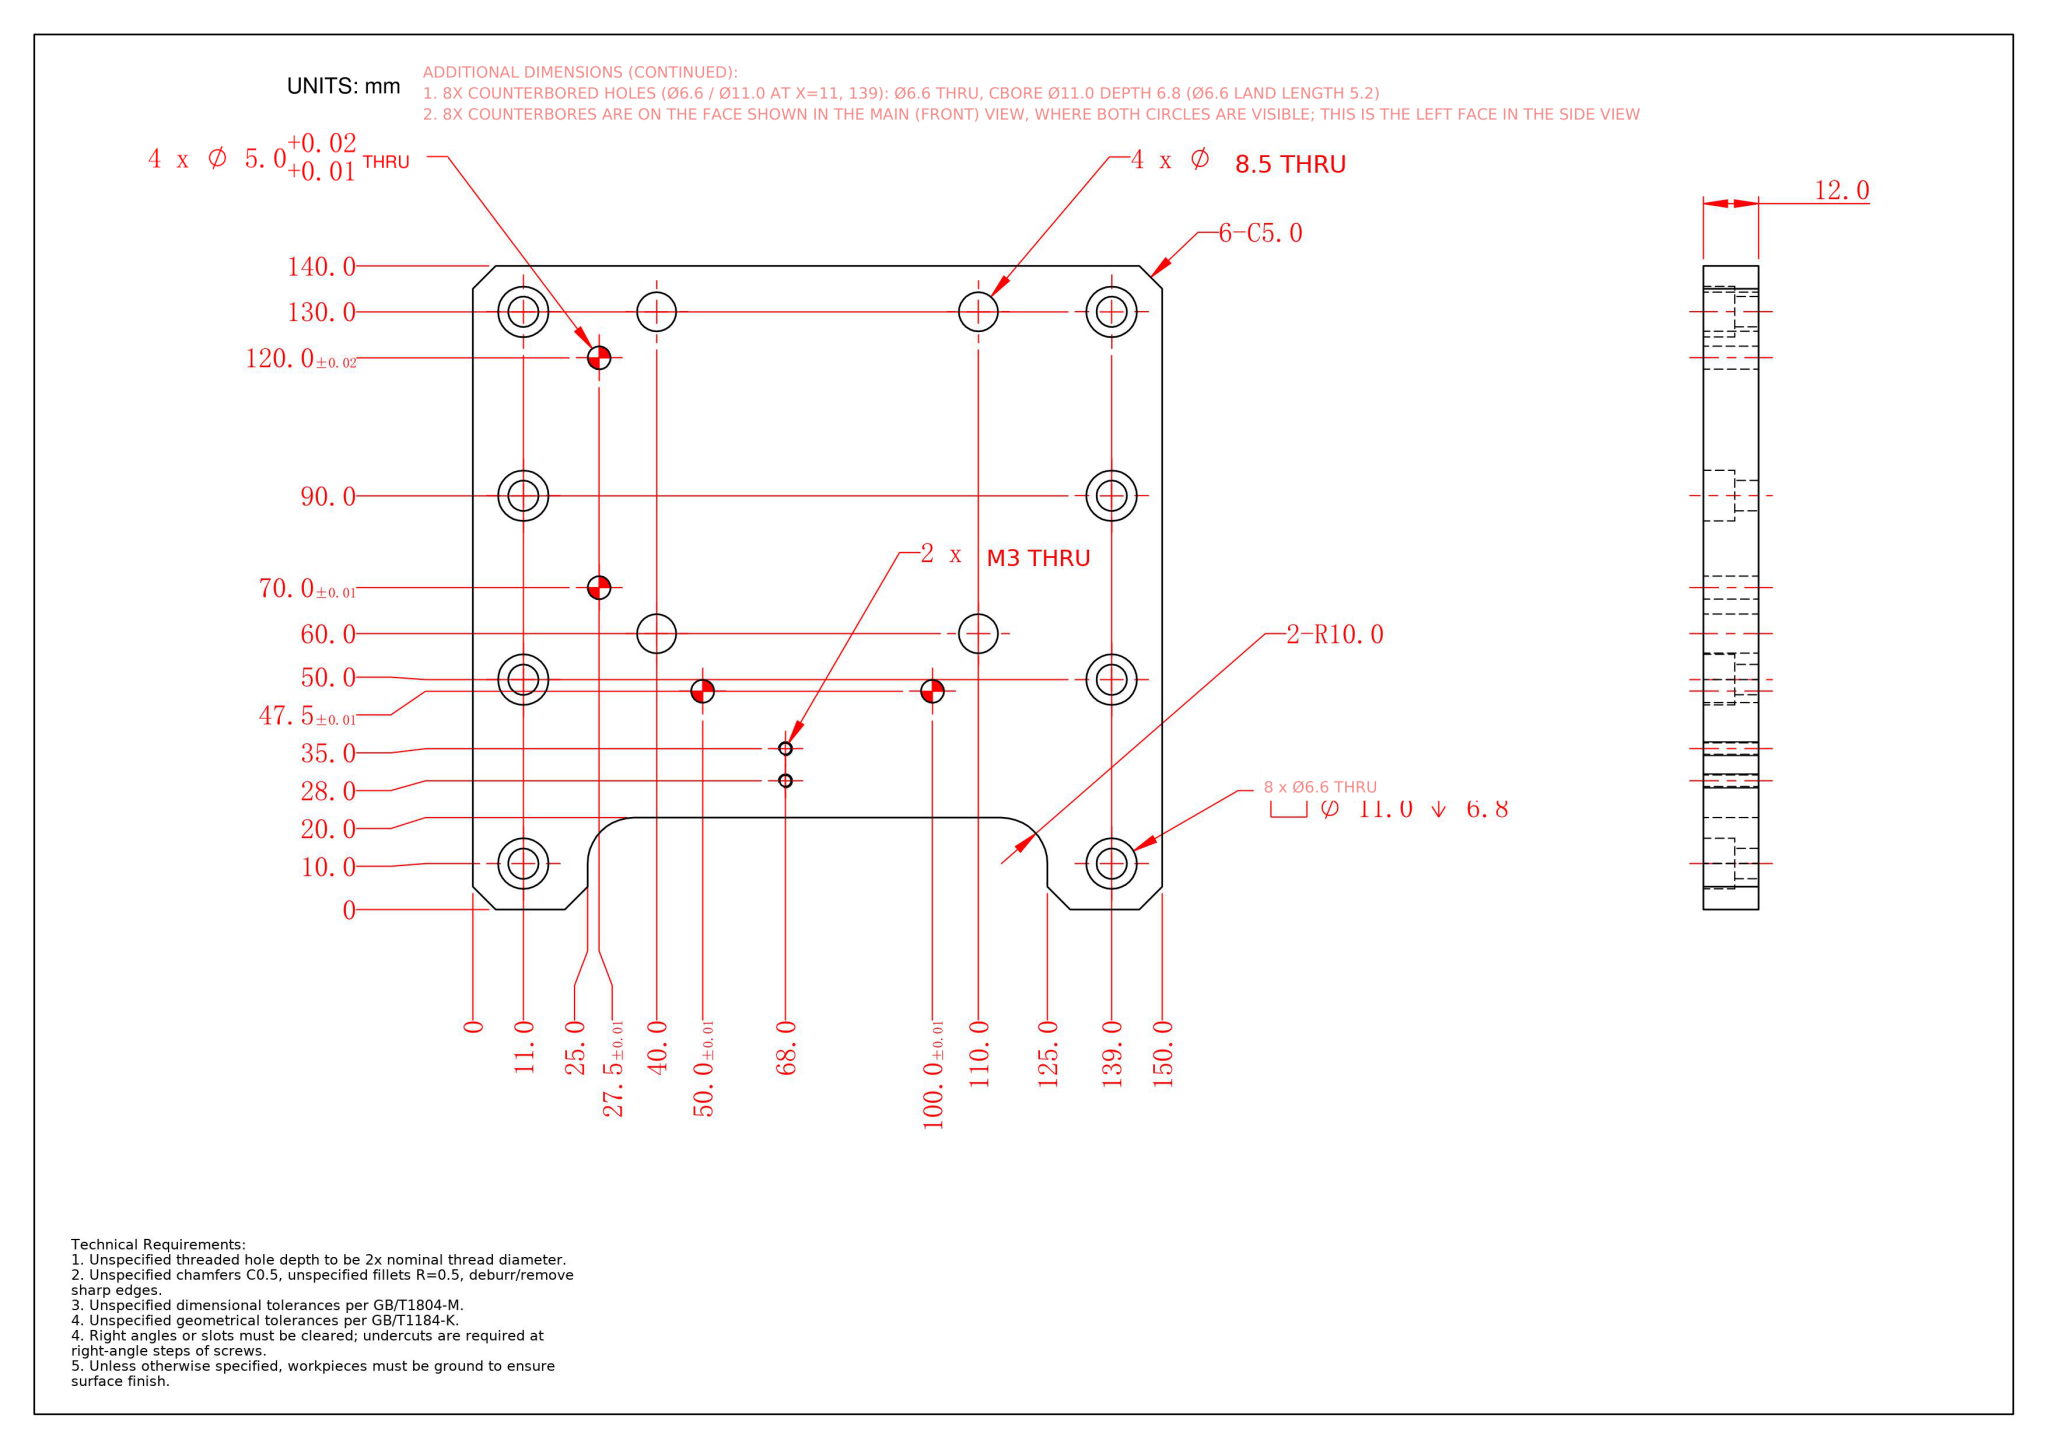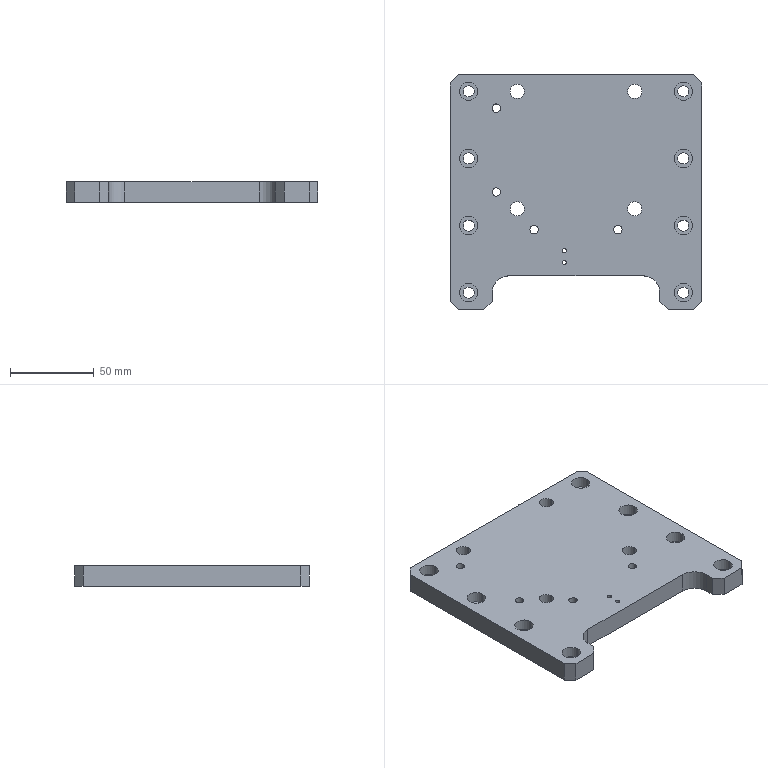Part | NX | mm | 1 solid | 78 faces | box 150 x 140 x 12 mm | volume 217238 mm3 | cylinder 54 | plane 24 | commonest cylinder face diameters 11 x16 6.6 x16 5 x8 8.5 x8 2.5 x4 20 x2